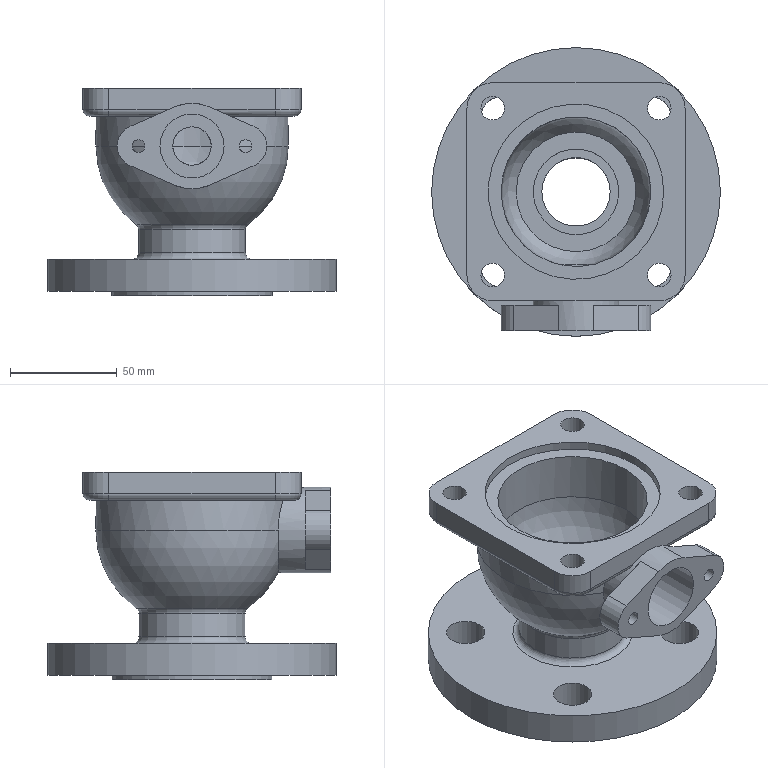Component | NX | VALVE_BODY | 1 solid | 60 faces | volume 433829 mm3 | cylinder 32 | plane 20 | torus 6 | sphere 2 | commonest cylinder face diameters 6 x7 18 x5 24 x4 11 x4 40 x2 20 x2 90 x1 82 x1